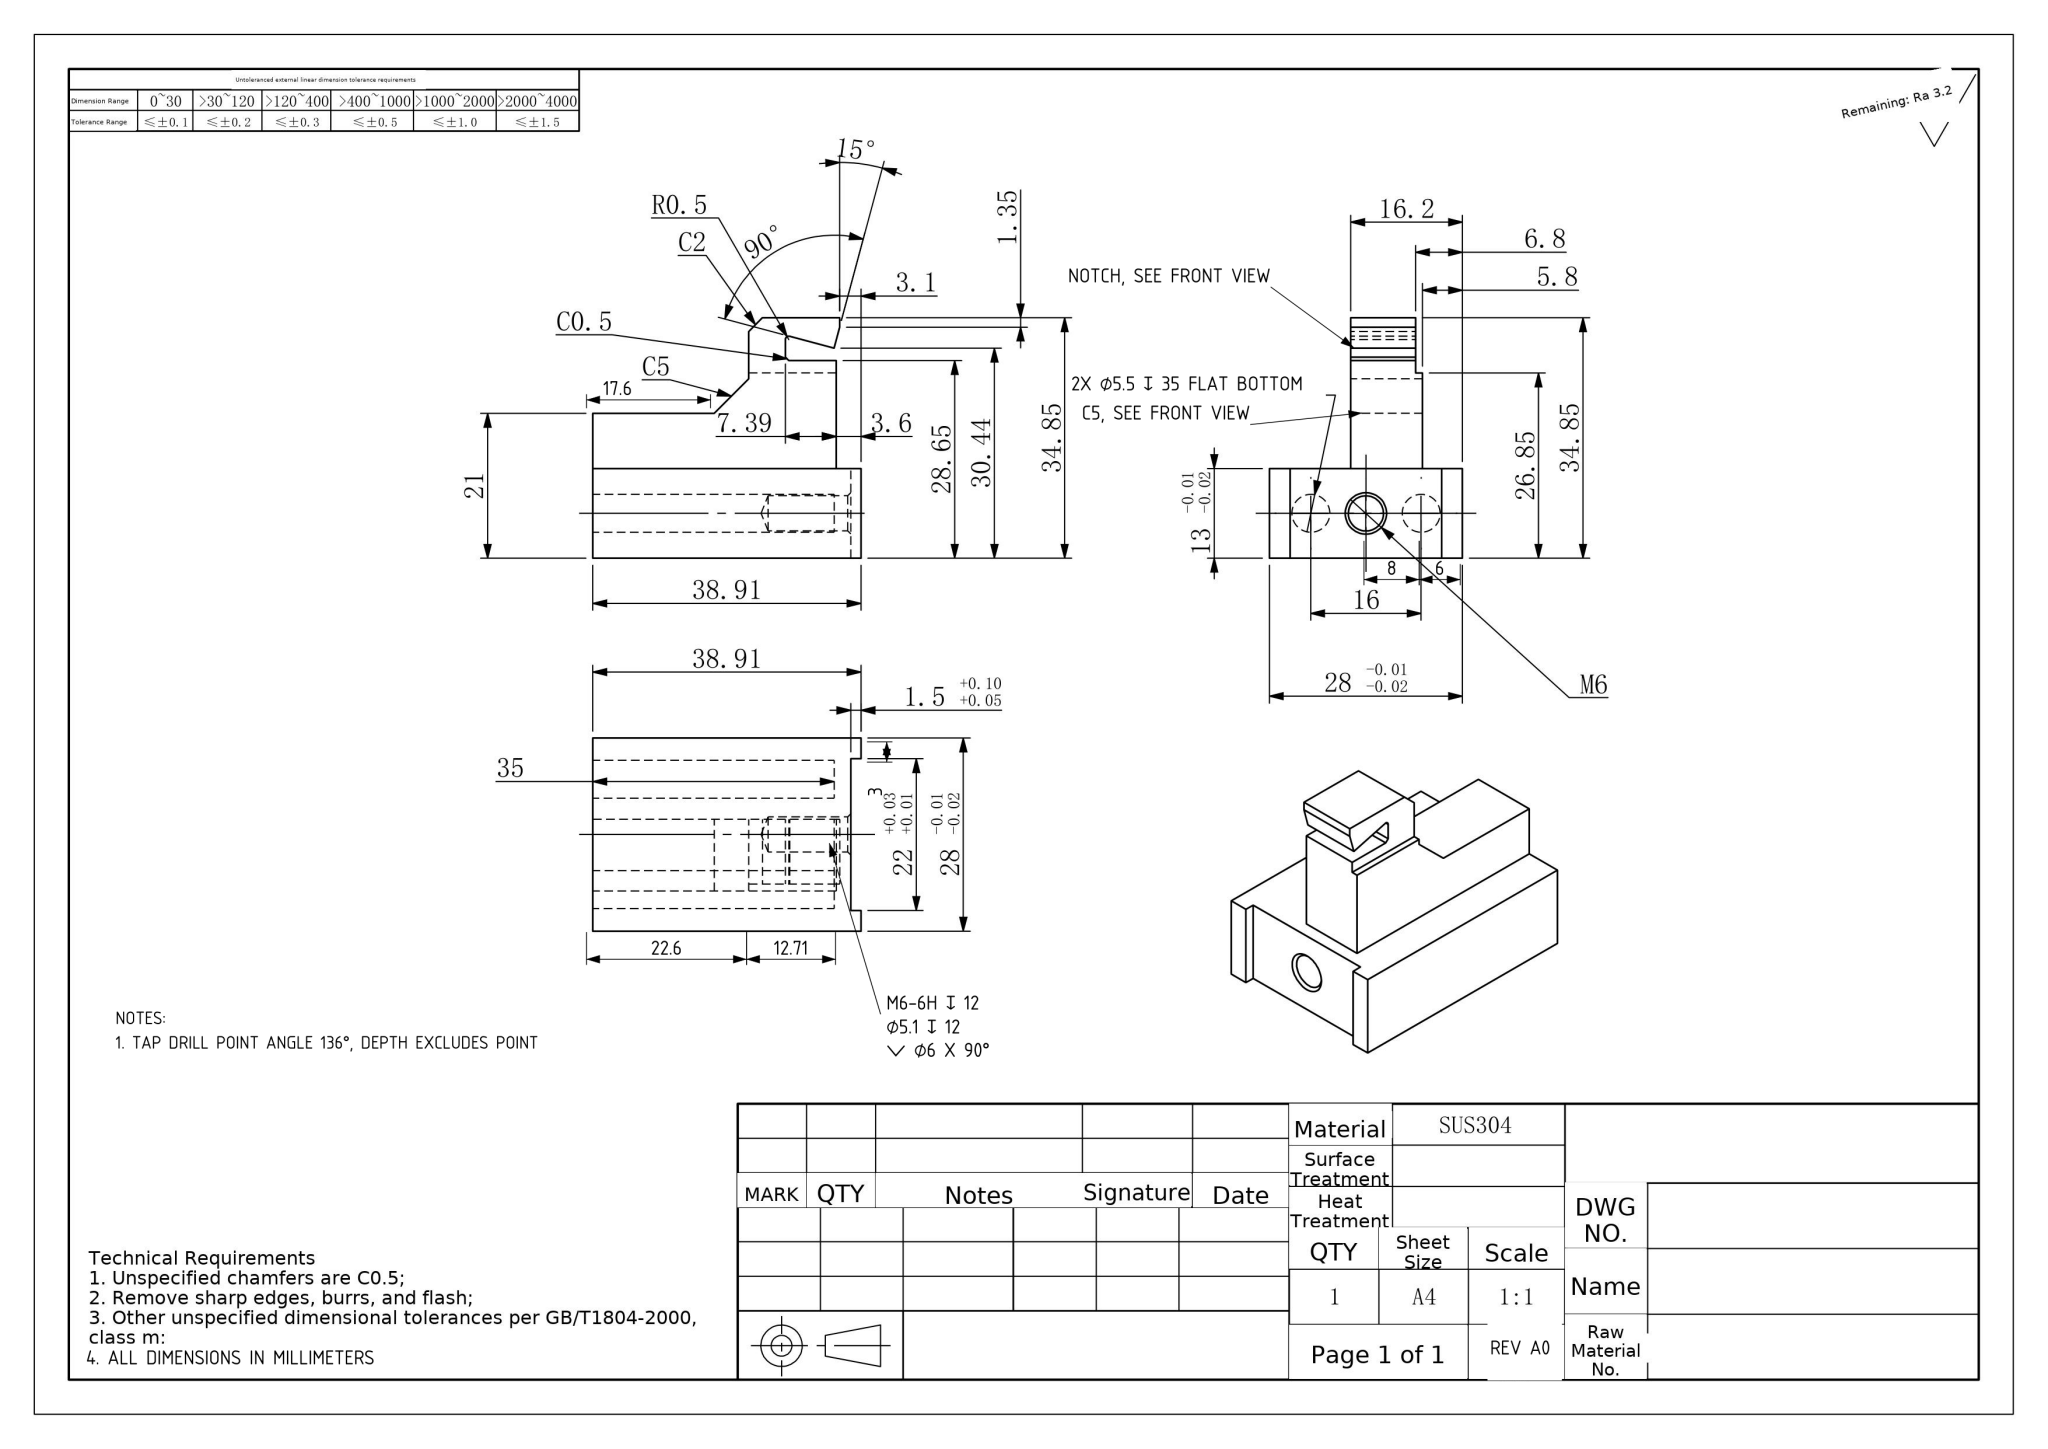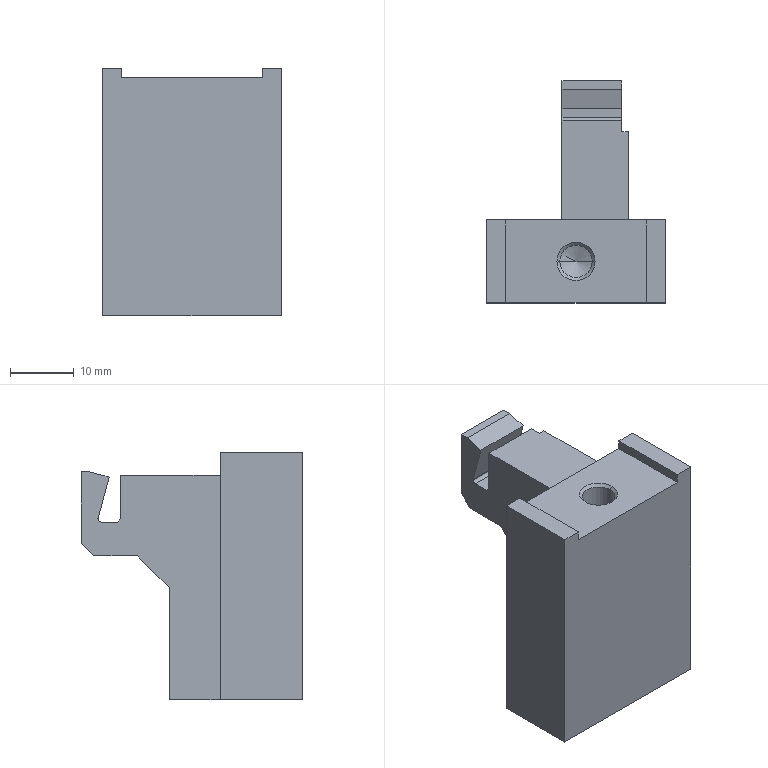Part | NX | mm | 1 solid | 40 faces | box 28 x 34.85 x 38.91 mm | volume 16418 mm3 | plane 28 | cylinder 8 | cone 4 | commonest cylinder face diameters 5.5 x4 1 x2 5.1 x2